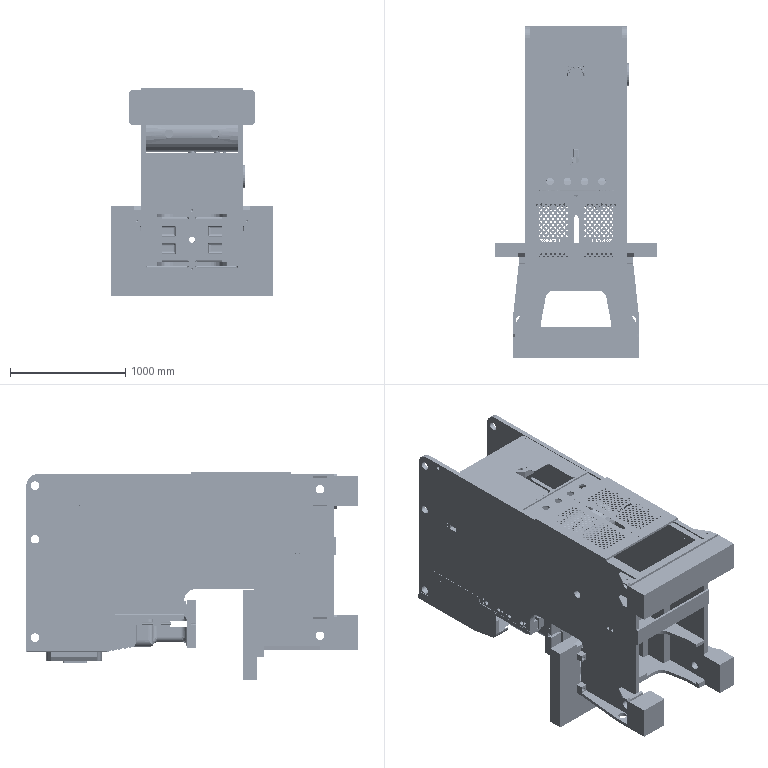Assembly | SolidWorks | mm | 131 component files | 131 solids | 7886 faces | box 1400 x 2883 x 1810 mm | volume 817598501 mm3 | plane 3870 | cylinder 2630 | cone 812 | spline 326 | torus 146 | sphere 102 | commonest cylinder face diameters 6 x283 13.5 x168 10 x153 1 x148 7 x146 5 x132 6.8 x98 17.5 x88
Bill of materials:
'-1_JF21-80.1-14-1-SOLID1 | 1 |  | Long, thin flat rectangular plate strip with a pattern of small through holes along both long edges and a few slightly larger holes near each end.
'-1_JF21-80.1-14-1-SOLID1-1 | 1 |  | Long thin flat plate strip with shallow rectangular pockets (or raised pads) in a staggered pattern down its length, plus through holes at the corners, along the edges and near the ends.
'-1_JF21-80.1-15-1-1-SOLID1 | 1 |  | Long flat bar with shallow stepped rectangular pockets or pads down its length. It has pairs of holes at both ends, holes spaced along the bar and small holes inside the end pockets.
'-1_JF21-80.1-15-1-1-SOLID1-1 | 1 |  | Long flat bar with shallow stepped rectangular pockets or pads down its length. It has pairs of holes at both ends, holes spaced along the bar and small holes inside the end pockets.
'-1_JF21-80.1-17-1-SOLID1 | 1 |  | Long inverted-T profile bar: a wide base flange with an upright web. It has small chamfered edges, larger through holes in the web and the base, and many small holes.
'-1_JF21-80.1-24-1-SOLID1 | 1 |  | Long inverted-T profile bar similar to the previous T-section part. It has three holes through the web, five larger holes in the base flange and very few small holes.
1 | 1 |  | Two-plate bracket. A thick rectangular vertical plate has rectangular slot-like pockets or windows, a central round hole and small corner holes. A thin horizontal plate is joined at right angles; it has a tapered outline, a large rounded U-shaped cutout and two mounting holes.
'-1-SOLID1 | 1 |  | L-shaped angle bracket: a flat rectangular top plate with a perpendicular leg along one edge. The leg has a vertical obround slot.
200TonPunchPress3DDrawing.sldasm-Part-1 | 1 |  | Thin square frame: a flat ring of constant width and thickness with a large square central opening.
'-2-SOLID1 | 1 |  | L-shaped angle bracket: a flat rectangular plate with a perpendicular leg along one edge. The leg has a vertical obround slot.
'-3[1] | 1 |  | Solid rectangular block with a rebate step along one lower edge, a narrow step or groove along the top rear edge, and a chamfered corner.
'-3[2] | 1 |  | Solid rectangular block with an L-shaped stepped footprint and a small notch or chamfer at one top corner.
'-3[3] | 1 |  | Long straight bar with a rectangular cross-section and a narrow bevel along one top long edge; the corners of the top-view outline are chamfered.
'-3-SOLID1 | 1 |  | L-shaped angle bracket made from constant-thickness plate, with one rounded-end (obround) slot through one leg.
'-4-SOLID1 | 1 |  | L-shaped angle bracket made from constant-thickness plate, with one obround slot through the vertical leg.
JF21-110.1-33-1-SOLID1 | 1 |  | Flat annular ring with a large central bore and four small through-holes spaced evenly on a bolt circle.
JF21-110.1-34-1-SOLID1 | 1 |  | Plain solid circular disc of uniform thickness with no visible holes or features.
JF21-110.2-20-1-SOLID1 | 1 |  | Long hollow cylindrical tube with a concentric through-bore and flat, square-cut ends.
JF21-63.1-17-1-SOLID1 | 1 |  | Solid cylindrical pin or rod with small chamfers at both ends.
JF21-63.1-17-2-SOLID1 | 1 |  | Solid cylindrical pin or rod with small chamfers at both ends.
JF21-63.1-24-1-SOLID1 | 1 |  | Rectangular block with a large cylindrical through-bore and a thin slit running from the bore to one side face (split-clamp style). Four through-holes run perpendicular to the bore.
JF21-63.1-24-2-SOLID1 | 1 |  | Rectangular block with a large cylindrical through-bore and a thin slit running from the bore to one side face. Four through-holes run perpendicular to the bore.
JF21-80.1.3-1-1-SOLID1 | 1 |  | Thin flat sheet plate, roughly square with rounded corners, with a stepped rectangular notch cut in from one edge. It has two keyhole slots near two corners and two small round holes near the opposite corners.
JF21-80.1-11-1-SOLID1 | 1 |  | Thin-walled cylindrical sleeve with chamfered ends, an external circumferential groove near one end, a small radial hole within that groove, and short axial slots at the rim. An internal step and an internal axial groove line are visible.
JF21-80.1-1-3(_)-1-SOLID10 | 1 |  | Short solid cylindrical disc with a small concentric through-bore; axial length less than outer diameter.
JF21-80.1-1-3(_)-1-SOLID1 | 1 |  | Long thin-walled open cylindrical tube with several round radial holes through the wall.
JF21-80.1-1-3(_)-1-SOLID11 | 1 |  | Short solid cylindrical disc with a small concentric through-bore; axial length less than outer diameter.
JF21-80.1-1-3(_)-1-SOLID12 | 1 |  | Cylindrical bushing/spacer-like ring with a concentric through-bore of moderate size; height roughly half the outer diameter.
JF21-80.1-1-3(_)-1-SOLID13 | 1 |  | Tall cylindrical sleeve with a concentric through-bore; height is close to the outer diameter.
JF21-80.1-1-3(_)-1-SOLID14 | 1 |  | Cylindrical ring/spacer with a larger concentric through-bore; height about half the outer diameter.
JF21-80.1-1-3(_)-1-SOLID15 | 1 |  | Thick-walled cylindrical ring/spacer with a large concentric through-bore; height about half the outer diameter.
JF21-80.1-1-3(_)-1-SOLID16 | 1 |  | Long, thin, flat rectangular bar with a single step in width partway along its length.
JF21-80.1-1-3(_)-1-SOLID17 | 1 |  | Flat plate of constant thickness, cut to an inverted-L outline: a long arm with a shorter leg at one end, a rounded inner corner relief, and a curved step in the arm's lower edge.
JF21-80.1-1-3(_)-1-SOLID18 | 1 |  | Flat plate of constant thickness, cut to an inverted-L outline: a long arm with a shorter leg at one end, a rounded inner corner relief, and a curved step in the arm's lower edge.
JF21-80.1-1-3(_)-1-SOLID19 | 1 |  | Thin rectangular plate/frame with rounded outer corners and a large central cutout made of one large circle merged with two smaller overlapping circular lobes, plus eight small through-holes near the edges.
JF21-80.1-1-3(_)-1-SOLID20 | 1 |  | Thick rectangular plate with a through-cutout of one large circle merged with two smaller overlapping circular lobes, a small hole near the cutout, and a trapezoidal tab with angled sides sticking out from one edge.
JF21-80.1-1-3(_)-1-SOLID2 | 1 |  | Thin flat circular disc of uniform thickness with no visible holes or features.
JF21-80.1-1-3(_)-1-SOLID21 | 1 |  | Thick annular ring (washer or spacer-like shape) with a concentric through-bore and one flat cut on the outer cylindrical edge.
JF21-80.1-1-3(_)-1-SOLID22 | 1 |  | Prismatic block with a constant cross-section: one corner has a concave quarter-round cutout, and the opposite side is a long angled (chamfer-like) face, so the profile is roughly a trapezoid.
JF21-80.1-1-3(_)-1-SOLID23 | 1 |  | Prismatic block with a concave quarter-round groove along one top edge and an angled side face that tapers the profile.
JF21-80.1-1-3(_)-1-SOLID24 | 1 |  | Prismatic block with a constant cross-section: a concave quarter-round cutout at one top corner and a large inclined face on the opposite lower side.
JF21-80.1-1-3(_)-1-SOLID25 | 1 |  | Prismatic block with a concave quarter-round cutout along one edge and an inclined face, giving a tapered profile.
JF21-80.1-1-3(_)-1-SOLID26 | 1 |  | Prismatic block with a tapered or skewed profile and a concave quarter-round cutout at one top corner. In the isometric view this cutout appears small relative to the block.
JF21-80.1-1-3(_)-1-SOLID27 | 1 |  | Thick cylindrical ring (bushing or spacer-like shape) with a concentric through-bore and one small radial hole through the outer wall.
JF21-80.1-1-3(_)-1-SOLID28 | 1 |  | Thin-walled open circular arc band of rectangular cross-section, roughly semicircular or slightly larger, with a wall height much greater than its wall thickness.
JF21-80.1-1-3(_)-1-SOLID29 | 1 |  | Thin flat open circular arc strip of rectangular cross-section, roughly semicircular or slightly larger, low in height compared to its radial width.
JF21-80.1-1-3(_)-1-SOLID30 | 1 |  | Long straight bar with a small rectangular cross-section and square-cut ends.
JF21-80.1-1-3(_)-1-SOLID3 | 1 |  | Thin flat circular disc of uniform thickness with no visible holes or features.
JF21-80.1-1-3(_)-1-SOLID31 | 1 |  | Thick annular ring (flange-like) with a large central bore and six small holes evenly spaced on a bolt circle; a narrow step or groove near the outer edge of the top face, and a local stepped/protruding feature on part of the underside.
JF21-80.1-1-3(_)-1-SOLID32 | 1 |  | Thin flat plate with a T-shaped outline: a wider strip along one edge over a narrower rectangular body, with one small round through hole offset toward one side.
JF21-80.1-1-3(_)-1-SOLID34 | 1 |  | Thin flat plate with a stepped outer outline and a large U-shaped cutout open at one edge; the cutout has rounded inner corners and sides that taper outward slightly toward the open end, leaving two legs.
JF21-80.1-1-3(_)-1-SOLID38 | 1 |  | Plain thin rectangular flat bar or strip with no visible holes or features.
JF21-80.1-1-3(_)-1-SOLID39 | 1 |  | Flat plate with a five-sided outline: a rectangle with one corner cut off by a long angled edge. No holes.
JF21-80.1-1-3(_)-1-SOLID40 | 1 |  | Flat plate with a five-sided outline: a rectangle with one corner cut off by a long angled edge (mirror orientation relative to unnamed part). No holes.
JF21-80.1-1-3(_)-1-SOLID4 | 1 |  | Very thin circular disc with no visible holes or features.
JF21-80.1-1-3(_)-1-SOLID41 | 1 |  | Flat plate with a five-sided outline: a rectangle with one corner cut off by an angled edge. No holes.
JF21-80.1-1-3(_)-1-SOLID42 | 1 |  | Flat plate with a five-sided outline (a rectangle with one angled corner cut) and one round through hole in the wider part of the plate.
JF21-80.1-1-3(_)-1-SOLID43 | 1 |  | Flat plate with a five-sided outline (a rectangle with one angled corner cut, mirrored relative to unnamed part) and one round through hole.
JF21-80.1-1-3(_)-1-SOLID44 | 1 |  | Cube-shaped block with a single large round through hole centered on one pair of opposite faces.
JF21-80.1-1-3(_)-1-SOLID45 | 1 |  | Near-cube block with a single large round through hole, placed off-center toward one side on the faces it passes through.
JF21-80.1-1-3(_)-1-SOLID46 | 1 |  | Cube-like rectangular block with one large round through-hole on one face, set off-center toward one side.
JF21-80.1-1-3(_)-1-SOLID47 | 1 |  | Cube-like rectangular block with one large round through-hole on one face, set off-center toward the side opposite to part-56fda0ee.
JF21-80.1-1-3(_)-1-SOLID48 | 1 |  | Cube-like rectangular block with one large off-center round through-hole; looks the same as part-af3b9697.
JF21-80.1-1-3(_)-1-SOLID49 | 1 |  | Thin flat rectangular plate with one small round through-hole near the middle of one long edge.
JF21-80.1-1-3(_)-1-SOLID50 | 1 |  | Square block, thinner than it is wide, with a large central round through-hole running through its thickness.
JF21-80.1-1-3(_)-1-SOLID5 | 1 |  | Thick cylindrical ring (short hollow cylinder) with a central round through-bore.
JF21-80.1-1-3(_)-1-SOLID51 | 1 |  | Thin flat plate, roughly rectangular, with a rectangular notch cut into the middle of each short end and one small round hole near one corner.
JF21-80.1-1-3(_)-1-SOLID52 | 1 |  | Long straight thin-walled C-shaped (channel) profile with a web and two parallel flanges, constant along its length.
JF21-80.1-1-3(_)-1-SOLID53 | 1 |  | Rectangular block with one round through-hole on the large face, set off-center toward one side.
JF21-80.1-1-3(_)-1-SOLID54 | 1 |  | Rectangular block with one off-center round through-hole; looks the same as part-8c164298.
JF21-80.1-1-3(_)-1-SOLID55 | 1 |  | Rectangular block with one round through-hole on the large face, set off-center toward the side opposite to part-8c164298.
JF21-80.1-1-3(_)-1-SOLID56 | 1 |  | Rectangular block with one off-center round through-hole; looks the same as part-ea095bbc.
JF21-80.1-1-3(_)-1-SOLID57 | 1 |  | Rectangular block with one vertical corner chamfered, a large through bore with a chamfered or counterbored edge, two small holes next to it, and a shallow narrow step along one top edge.
JF21-80.1-1-3(_)-1-SOLID58 | 1 |  | Rectangular block with one vertical corner chamfered, a large through bore with a chamfered or counterbored edge, two small holes next to it, and a narrow step or rabbet along one top edge.
JF21-80.1-1-3(_)-1-SOLID59 | 1 |  | Thick annular ring with a large central bore and six small holes evenly spaced around the face. It has a stepped outer profile with a raised or offset section on one side.
JF21-80.1-1-3(_)-1-SOLID60 | 1 |  | Plain straight bar with a square cross-section and flat ends.
JF21-80.1-1-3(_)-1-SOLID6 | 1 |  | Thick cylindrical spacer or bushing-like ring with a central through bore.
JF21-80.1-1-3(_)-1-SOLID61 | 1 |  | Plain straight bar with a square cross-section and flat ends.
JF21-80.1-1-3(_)-1-SOLID62 | 1 |  | Flat rectangular plate tab with one corner chamfered at one end and a single round through hole near the other end.
JF21-80.1-1-3(_)-1-SOLID63 | 1 |  | Flat rectangular plate tab with one chamfered corner and a single round through hole near the opposite end.
JF21-80.1-1-3(_)-1-SOLID64 | 1 |  | Flat rectangular plate tab with one chamfered corner and a single round through hole near the opposite end.
JF21-80.1-1-3(_)-1-SOLID65 | 1 |  | Flat rectangular plate tab with one chamfered corner and a single round through hole near the opposite end.
JF21-80.1-1-3(_)-1-SOLID66 | 1 |  | Long, thin rectangular bar with a shallow step along one long edge, giving a stepped or rabbeted profile.
JF21-80.1-1-3(_)-1-SOLID67 | 1 |  | Long thin plate with a thickened lip along one long edge (L-shaped end profile) and eleven round through holes in groups: three at each end and four in the middle, in two sizes.
JF21-80.1-1-3(_)-1-SOLID68 | 1 |  | Thin flat U-shaped plate frame: two long parallel arms joined by a wider cross bar with four equally spaced round through-holes in a row; inner corners of the opening are rounded.
JF21-80.1-1-3(_)-1-SOLID69 | 1 |  | Long rectangular bar with a stepped (rebated) cross-section that leaves a thicker lip along one long edge. It has ten round through-holes: a cluster of three near each end (two smaller and one larger) and four near the middle (two larger outer and two smaller inner).
JF21-80.1-1-3(_)-1-SOLID70 | 1 |  | Long angle-section (L-profile) strip with a joggle: the middle section is offset from the two end sections by short angled transitions.
JF21-80.1-1-3(_)-1-SOLID7 | 1 |  | Thick cylindrical ring or spacer with a central round through-bore. The outer diameter is about 2.5-3 times the bore diameter, and the height is a little under half the outer diameter.
JF21-80.1-1-3(_)-1-SOLID71 | 1 |  | Solid flat plate with a five-sided outline: a rectangle with one corner cut off by a long straight angled edge. No holes are visible.
JF21-80.1-1-3(_)-1-SOLID72 | 1 |  | Thin flat plate: roughly square, with a narrower stepped tab section at one end. It has two round through-holes of different sizes. The smaller hole lies in the tab and has a flat chord on the side toward the edge.
JF21-80.1-1-3(_)-1-SOLID73 | 1 |  | Thin rectangular plate with one rounded corner and a large stepped rectangular notch cut into one long edge. Features include corner and edge mounting holes, a long narrow slot, a larger round hole, and several groups of very small holes.
JF21-80.1-1-3(_)-1-SOLID74 | 1 |  | Flat rectangular plate with one large round through-hole and one smaller round through-hole on the centerline. The smaller hole has four small holes arranged around it, and a faint circular outline appears around it on one face.
JF21-80.1-1-3(_)-1-SOLID75 | 1 |  | Thin rectangular plate with one rounded corner and a stepped rectangular notch in one long edge. It has perimeter mounting holes, one interior round hole, a small rectangular cutout with tiny marks beside it, and rows of very small holes.
JF21-80.1-1-3(_)-1-SOLID76 | 1 |  | Plain solid right circular cylinder with flat ends. Diameter is roughly 1.6-1.8 times the height. No holes or other features are visible.
JF21-80.1-1-3(_)-1-SOLID77 | 1 |  | Plain solid right circular cylinder with flat ends. Diameter is roughly 1.6-1.8 times the height. No holes or other features are visible.
JF21-80.1-1-3(_)-1-SOLID78 | 1 |  | Plain solid right circular cylinder with flat ends. Diameter is roughly 1.6-1.8 times the height. No holes or other features are visible.
JF21-80.1-1-3(_)-1-SOLID79 | 1 |  | Solid plain cylinder (puck/short rod) with flat parallel end faces and no visible holes or features.
JF21-80.1-1-3(_)-1-SOLID8 | 1 |  | Thick-walled cylindrical sleeve/spacer with a central through bore.
JF21-80.1-1-3(_)-1-SOLID9 | 1 |  | Thick-walled cylindrical sleeve/spacer with a central through bore; looks the same as unnamed part.
JF21-80.1-13-1-SOLID1 | 1 |  | Long thin flat strip with rounded corners and five evenly spaced semicircular open notches along one long edge (including near each end).
JF21-80.1-16-1-SOLID1 | 1 |  | Long flat rectangular bar/plate with a row of larger through holes along the centerline and smaller through holes staggered on alternate sides; the ends have one large hole with two small holes beside it.
JF21-80.1-16-2-SOLID1 | 1 |  | Long flat perforated bar with larger centerline holes, smaller staggered holes, and small-hole clusters at the ends; looks the same as unnamed part.
JF21-80.1-18-1-SOLID1 | 1 |  | Long thin flat strip with rounded corners and five evenly spaced semicircular open notches along one long edge; this is the opposite edge compared with unnamed part.
JF21-80.1-20-1-SOLID1 | 1 |  | Long rectangular bar with chamfered long edges (octagon-like cross-section), a row of seven through holes along the top face, a few tiny point marks, and one transverse hole through the side near one end.
JF21-80.1-20-2-SOLID1 | 1 |  | Long rectangular bar with chamfered long edges, seven top-face holes along the centerline, tiny point marks, and one side hole near one end; looks the same as unnamed part.
JF21-80.1-30-1-SOLID1 | 1 |  | Solid circular disc (blind-flange-like plate) with six evenly spaced through holes on a bolt circle and a shallow raised, smaller-diameter face on one side.
JF21-80.1-33-1-SOLID1 | 1 |  | Very thin flat annular ring with a large central opening and six evenly spaced holes on a bolt circle.
JF21-80.2-12-1-SOLID1 | 1 |  | Square base plate with rounded corners and a raised cylindrical tubular boss with a large through bore. The boss has a circumferential groove near its top and an annular recess/groove in its top face; there are small radial holes in the boss wall, four corner through holes, and two smaller diagonal holes in the plate.
JF21-80.2-13-1-SOLID1 | 1 |  | Thin circular disc with chamfered outer edges. The top face has a recessed pocket with concentric stepped rings, four through holes evenly spaced on a circle, and a small central through hole.
JF21-80.2-14-1-SOLID1 | 1 |  | Thin, flat, tapered plate shaped like a teardrop. One end is rounded and has a single circular through hole; the plate narrows to a small squared-off tip at the other end.
JF21-80.2-32A-1-SOLID1 | 1 |  | Annular ring with a thick cylindrical base and a large central bore. A smaller-diameter stepped collar rises from the top and has a circumferential groove. Six small holes are evenly spaced around the outer flange face.
JF21-80.2-34-1-SOLID1 | 1 |  | Thin bent bracket with a flat main plate and one edge folded about 90 degrees into a flange. The flat portion is a trapezoid-like shape with rounded lobes and four circular through holes: three along the wide edge and one near the narrow end.
JF21-80.2-40-1-SOLID10 | 1 |  | Plain solid rectangular bar (cuboid) with no visible holes or features.
JF21-80.2-40-1-SOLID1 | 1 |  | Square flat plate with rounded corners, a small through hole near each corner, and a larger central through hole.
JF21-80.2-40-1-SOLID11 | 1 |  | Plain solid rectangular bar (cuboid) shown rotated in the views, with no visible holes or features.
JF21-80.2-40-1-SOLID12 | 1 |  | Plain solid rectangular bar (cuboid) with no visible features, oriented at an angle in the plan view.
JF21-80.2-40-1-SOLID13 | 1 |  | Plain solid rectangular bar (cuboid) with no visible features, oriented at an angle in the plan view.
JF21-80.2-40-1-SOLID14 | 1 |  | Plain solid rectangular bar (cuboid), relatively wide and flat, with no visible holes or features.
JF21-80.2-40-1-SOLID2 | 1 |  | Plain solid rectangular bar (cuboid) with no visible features, oriented at an angle in the plan view.
JF21-80.2-40-1-SOLID3 | 1 |  | Plain solid rectangular bar (cuboid) with no visible holes or features.
JF21-80.2-40-1-SOLID4 | 1 |  | Plain solid rectangular bar / block, elongated with a rectangular cross-section; no holes, chamfers, or other features visible.
JF21-80.2-40-1-SOLID5 | 1 |  | Plain solid rectangular bar / block, elongated with a rectangular cross-section; looks like the same simple prism shape as unnamed part, shown in a different orientation.
JF21-80.2-40-1-SOLID6 | 1 |  | Plain solid rectangular bar with a rectangular cross-section, shown rotated relative to the view axes; no features beyond the prism faces.
JF21-80.2-40-1-SOLID7 | 1 |  | Plain solid rectangular bar with a rectangular cross-section, shown rotated relative to the view axes; no holes or cut features.
JF21-80.2-40-1-SOLID8 | 1 |  | Plain solid rectangular bar with a rectangular cross-section, shown rotated relative to the view axes; no secondary features.
JF21-80.2-40-1-SOLID9 | 1 |  | Plain solid rectangular bar with a rectangular cross-section, shown rotated relative to the view axes; no holes or cut features.
JH21-80.1.4-1.1-1()()-1-SOLID1 | 1 |  | Thin-walled, bent-sheet-style U-channel tray / cradle. It has a flat base with a large central cutout (roughly rectangular, with arc-shaped ends) and two tall side walls with stepped, rounded outlines. Each side wall has two small through-holes. A shorter lip/flange at one end also has two small holes. The base has notches with sloped edges at one end, and the bottom edge of one end is angled.
JH21-80.1.4-1.2-2()()-1-SOLID1 | 1 |  | Thin-walled tray / cradle. It has a flat base with two straight side walls angled outward (chamfer-like bends near the floor) and two curved, arc-shaped end walls that are separate from the side walls, leaving gaps at the corners. The base has a pattern of five holes: one larger central hole surrounded by four smaller holes in a rectangle.
JH21-80.1.6-1()-1-SOLID1 | 1 |  | Thin flat plate, roughly rectangular, with rounded corners. One long edge has a wide, shallow notch with angled transitions. The plate has a dense array of small hexagonal perforations in two fields, separated by a band of cut-out lettering that reads 'YANGLI'.
JH21-80.1.6-1()-1-SOLID2 | 1 |  | Thin flat perforated plate that looks like a mirror image of unnamed part. It is roughly rectangular, with a shallow notch with angled ends on the opposite long edge and rounded corners. Hexagonal perforations sit in two fields, with cut-out lettering between them that appears mirrored in the views.
JZ21-80.4-1-1-SOLID1 | 1 |  | Complex machined-looking solid block / housing body. The top surface is flat, with a large U-shaped open notch at one end and two long shallow grooves running along it. One end has a thicker stepped section with pockets, short cylindrical bosses, a counterbored hole surrounded by a small hole pattern, and a rectangular recess. The underside has pockets and a side opening, and the profile tapers on one side. The end face has a large central through-hole, two cone-shaped recesses, crossing shallow grooves, and small holes at the four corners. Small keyhole-shaped slots appear along one edge.
Mates: